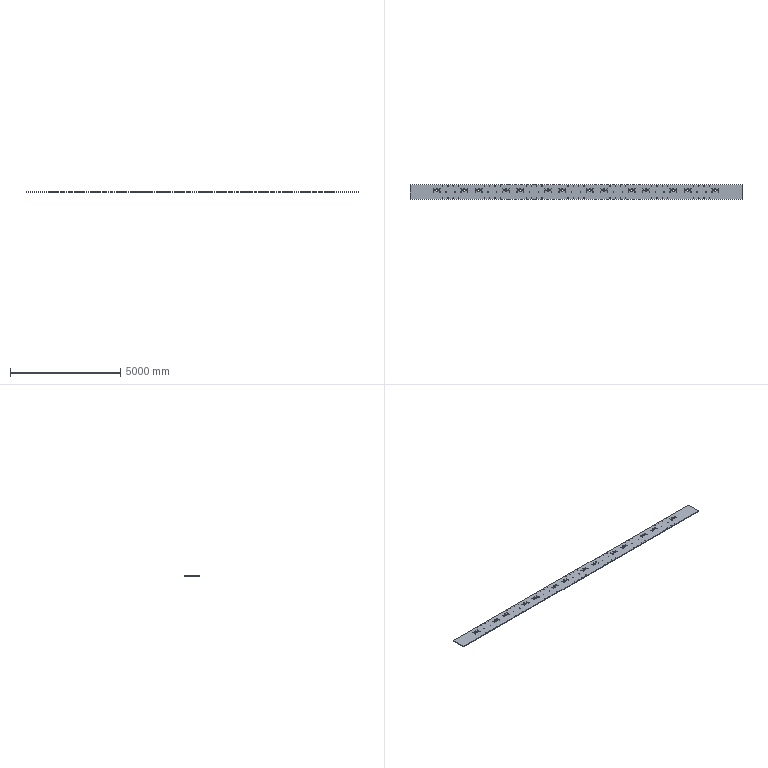Component | SolidWorks | ElectromagneticBeamBasePlate1-1 | 1 solid | 384 faces | volume 287967100 mm3 | cylinder 350 | plane 34 | commonest cylinder face diameters 14 x252 55 x56 90 x28 45 x14 | material Plain Carbon Steel